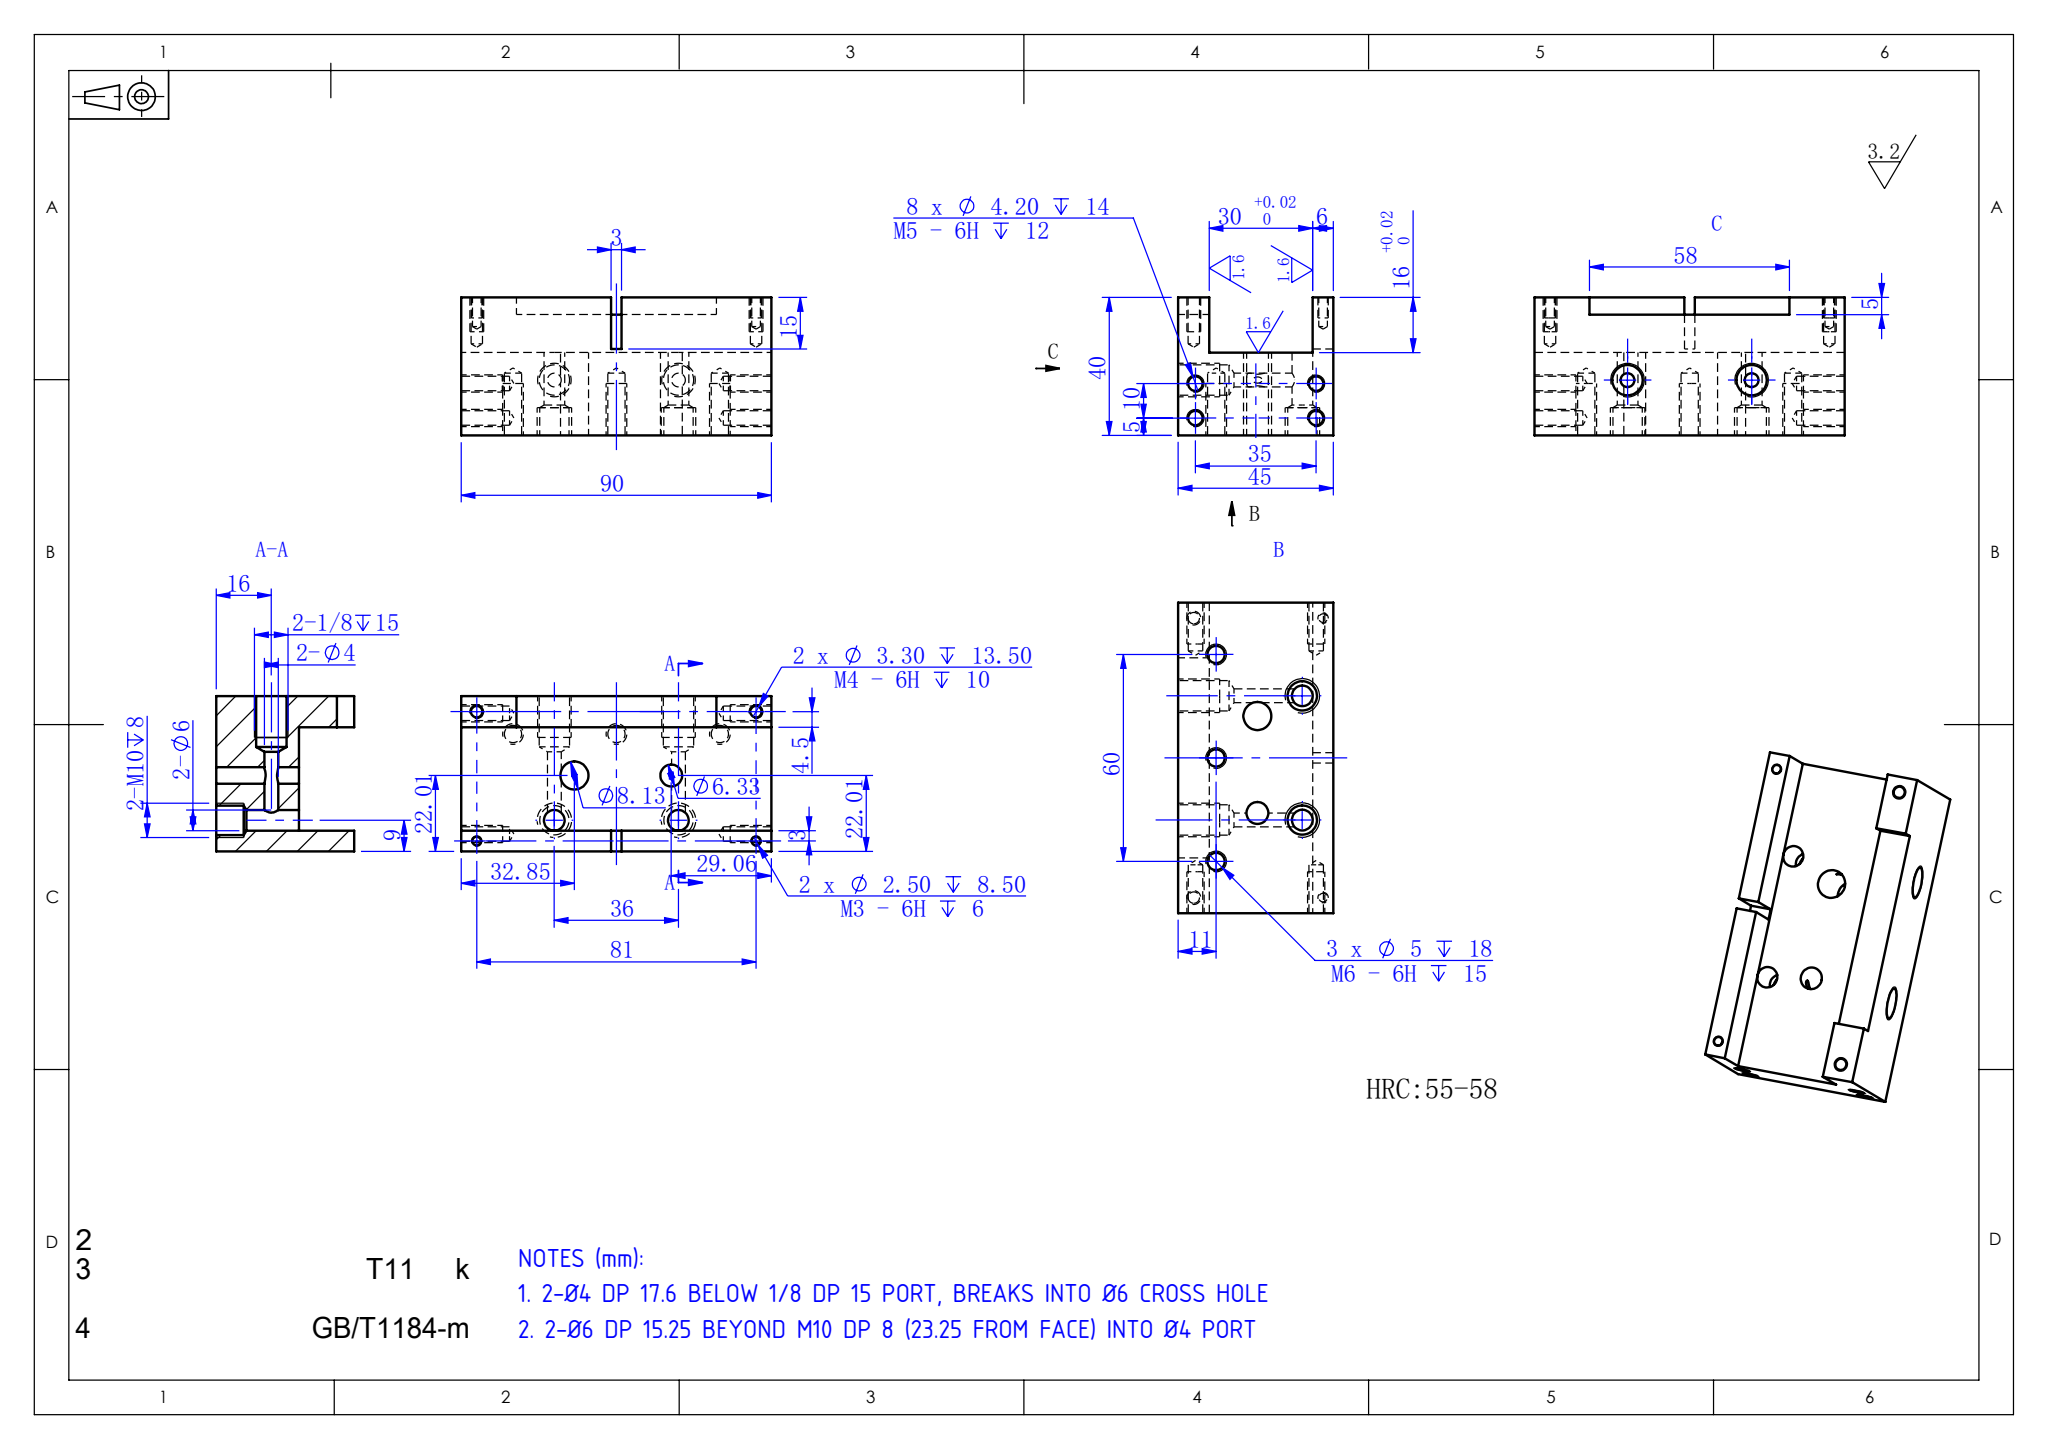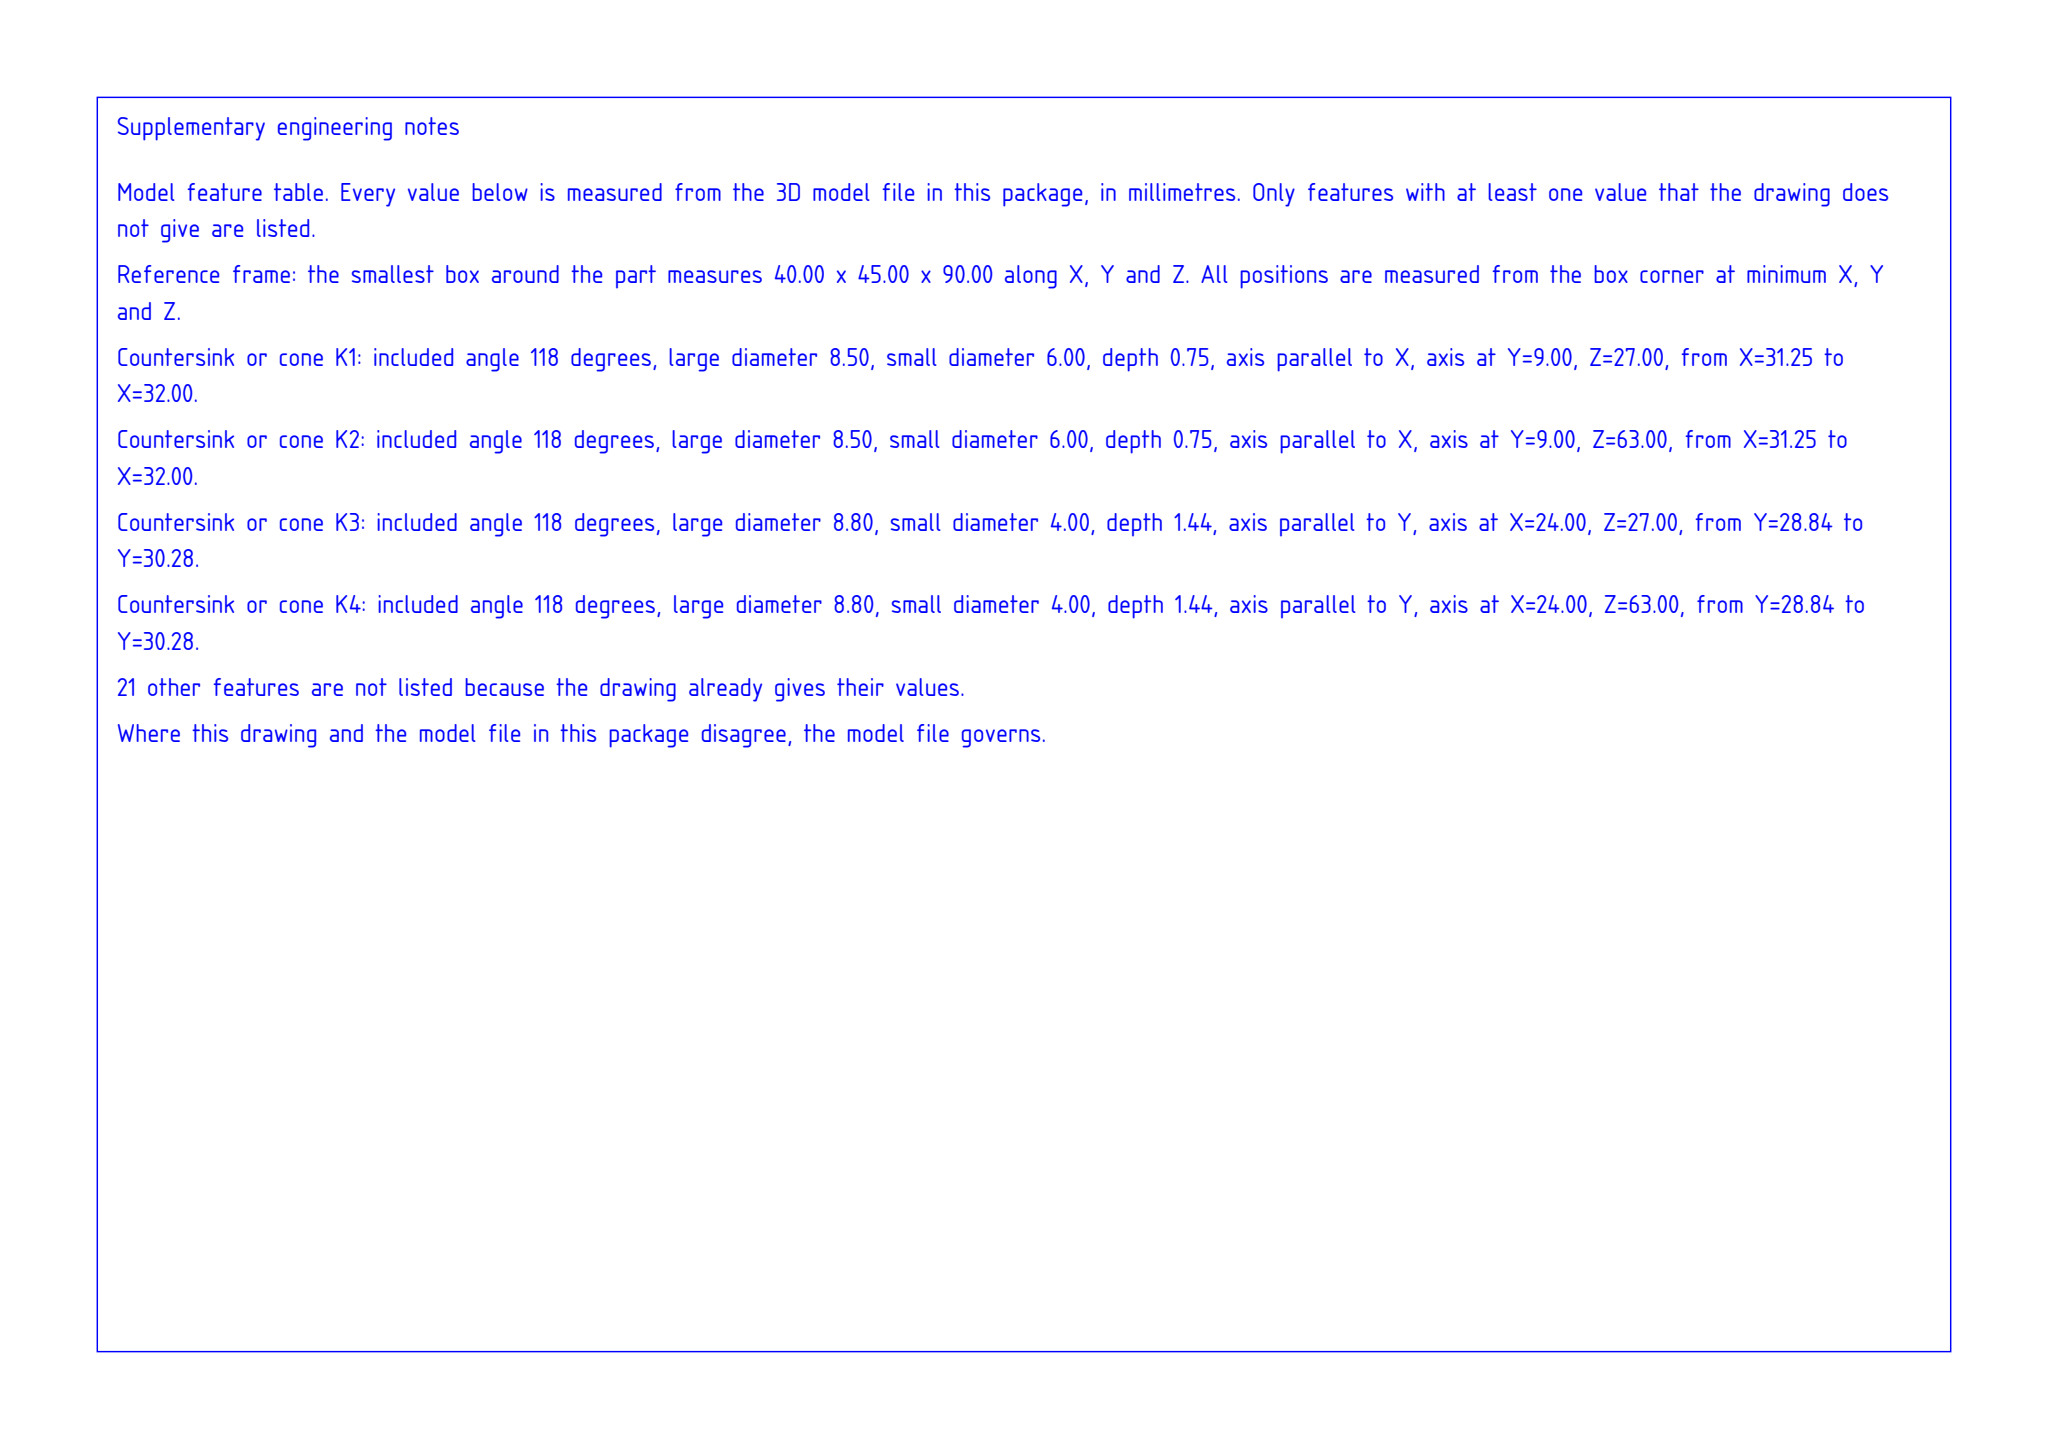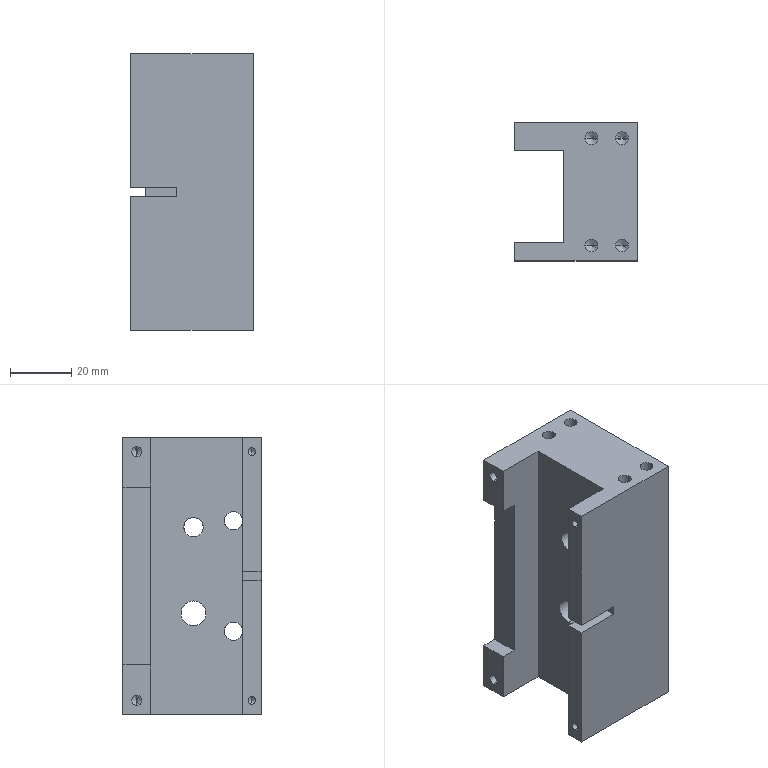Part | SolidWorks | mm | 1 solid | 106 faces | box 40 x 45 x 90 mm | volume 106811 mm3 | cylinder 50 | cone 38 | plane 18 | commonest cylinder face diameters 4.2 x16 5 x6 2.5 x4 3.3 x4 8.8 x4 4 x4 8.5 x4 6 x4
Drawing notes:
2-Ø4 DP 17.6 BELOW 1/8 DP 15 PORT, BREAKS INTO Ø6 CROSS HOLE | from the solid: cyl dia 4.0 axis y at x=24, z=27 & 63, length 17.6, below dia 8.8 y-hole (len 14.72) for 1/8 tap
2-Ø6 DP 15.25 BEYOND M10 DP 8 (23.25 FROM FACE) INTO Ø4 PORT | from the solid: cyl dia 6.0 axis x at y=9, z=27 & 63, length 15.25, following dia 8.5 x-hole length 8.0 from x=0 face; meets Ø4 at x=24
build123d program:
from build123d import *

# Parameters (mm, degrees)
SKETCH1_W                  = 40
SKETCH1_H                  = 45
BOSS_EXTRUDE1_DEPTH        = 90
SKETCH2_W                  = 16
SKETCH2_H                  = 30
CUT_EXTRUDE1_DEPTH         = 161.715
SKETCH3_W                  = 15
SKETCH3_H                  = 3
CUT_EXTRUDE2_DEPTH         = 6
SKETCH4_W                  = 58
SKETCH4_H                  = 9
CUT_EXTRUDE3_DEPTH         = 5
SKETCH5_R                  = 3
CUT_EXTRUDE4_DEPTH         = 107.791
M5_TAPPED_HOLE1_AT_2_COUNT = 2
M5_TAPPED_HOLE1_AT_2_PITCH = 35
M5_TAPPED_HOLE1_AT_3_COUNT = 2
M5_TAPPED_HOLE1_AT_3_PITCH = 36.401
M5_TAPPED_HOLE1_AT_4_COUNT = 2
M5_TAPPED_HOLE1_AT_4_PITCH = 10
M10_TAPPED_HOLE1_D         = 8.5
M10_TAPPED_HOLE1_DEPTH     = 8
M10_TAPPED_HOLE1_TIP       = 2.554
CUT_EXTRUDE6_REACH         = 160.512
SKETCH12_R                 = 2
G1_8_TAPPED_HOLE1_D        = 8.8
G1_8_TAPPED_HOLE1_DEPTH    = 14.72
G1_8_TAPPED_HOLE1_TIP      = 2.644
M4_TAPPED_HOLE1_D          = 3.3
M4_TAPPED_HOLE1_DEPTH      = 13.5
M4_TAPPED_HOLE1_TIP        = 0.9914
M3_TAPPED_HOLE1_D          = 2.5
M3_TAPPED_HOLE1_DEPTH      = 8.5
M3_TAPPED_HOLE1_TIP        = 0.7511
M6_TAPPED_HOLE1_D          = 5
M6_TAPPED_HOLE1_DEPTH      = 18
M6_TAPPED_HOLE1_TIP        = 1.502
SKETCH21_R                 = 3.165
SKETCH21_R_2               = 4.065
CUT_EXTRUDE7_DEPTH         = 62


with BuildPart() as part:
    # Sketch1 → Boss-Extrude1 (new body)
    with BuildSketch(Plane.XY):
        with Locations((-102.479, 29.734)):
            Rectangle(SKETCH1_W, SKETCH1_H)
    extrude(amount=BOSS_EXTRUDE1_DEPTH)

    # Sketch2 → Cut-Extrude1 (cut, through all)
    with BuildSketch(Plane.XY.offset(90)):
        with Locations((-114.479, 28.234)):
            Rectangle(SKETCH2_W, SKETCH2_H)
    extrude(amount=-CUT_EXTRUDE1_DEPTH, mode=Mode.SUBTRACT)

    # Sketch3 → Cut-Extrude2 (cut)
    with BuildSketch(Plane(origin=(0, 7.234, 0), x_dir=(-1, 0, 0), z_dir=(0, -1, 0))):
        with Locations((114.979, -45)):
            Rectangle(SKETCH3_W, SKETCH3_H)
    extrude(amount=-CUT_EXTRUDE2_DEPTH, mode=Mode.SUBTRACT)

    # Sketch4 → Cut-Extrude3 (cut)
    with BuildSketch(Plane.ZY.offset(122.479)):
        with Locations((45, 47.734)):
            Rectangle(SKETCH4_W, SKETCH4_H)
    extrude(amount=-CUT_EXTRUDE3_DEPTH, mode=Mode.SUBTRACT)

    # Sketch5 → Cut-Extrude4 (cut, through all)
    with BuildSketch(Plane.ZY.offset(106.479)):
        with Locations(Location((63, 16.234, 0), (0, 0, 270))):
            Circle(SKETCH5_R)
        with Locations(Location((27, 16.234, 0), (0, 0, 270))):
            Circle(SKETCH5_R)
    extrude(amount=-CUT_EXTRUDE4_DEPTH, mode=Mode.SUBTRACT)

    # Sketch6 → M5 Tapped Hole1 (revolve, cut)
    with BuildSketch(Plane(origin=(-97.479, 12.234, 90), x_dir=(0, -1, 0), z_dir=(1, 0, 0))):
        Polygon((0, 0), (0, 15.262), (2.1, 14), (2.1, 0), align=None)
    m5_tapped_hole1 = revolve(axis=Axis((-97.479, 12.234, 96.35), (0, 0, -1)), mode=Mode.SUBTRACT)

    # M5 Tapped Hole1 at 2: M5 Tapped Hole1 ×2
    with Locations(*[(0, i * M5_TAPPED_HOLE1_AT_2_PITCH, 0) for i in range(1, M5_TAPPED_HOLE1_AT_2_COUNT)]):
        add(m5_tapped_hole1, mode=Mode.SUBTRACT)

    # M5 Tapped Hole1 at 3: M5 Tapped Hole1 ×2
    with Locations(*[Vector(0.2747, 0.9615, 0) * (i * M5_TAPPED_HOLE1_AT_3_PITCH) for i in range(1, M5_TAPPED_HOLE1_AT_3_COUNT)]):
        add(m5_tapped_hole1, mode=Mode.SUBTRACT)

    # M5 Tapped Hole1 at 4: M5 Tapped Hole1 ×2
    with Locations(*[(i * M5_TAPPED_HOLE1_AT_4_PITCH, 0, 0) for i in range(1, M5_TAPPED_HOLE1_AT_4_COUNT)]):
        add(m5_tapped_hole1, mode=Mode.SUBTRACT)

    # Mirror1: M5 Tapped Hole1 across plane
    add(m5_tapped_hole1.mirror(Plane.XY.offset(45)), mode=Mode.SUBTRACT)

    # Mirror1 copy 1 sketch → Mirror1 copy 1 (revolve, cut)
    with BuildSketch(Plane(origin=(-97.479, 47.234, 0), x_dir=(0, -1, 0), z_dir=(1, 0, 0))):
        Polygon((0, 0), (0, -15.262), (2.1, -14), (2.1, 0), align=None)
    revolve(axis=Axis((-97.479, 47.234, -6.35), (0, 0, -1)), mode=Mode.SUBTRACT)

    # Mirror1 copy 2 sketch → Mirror1 copy 2 (revolve, cut)
    with BuildSketch(Plane(origin=(-87.479, 47.234, 0), x_dir=(0, -1, 0), z_dir=(1, 0, 0))):
        Polygon((0, 0), (0, -15.262), (2.1, -14), (2.1, 0), align=None)
    revolve(axis=Axis((-87.479, 47.234, -6.35), (0, 0, -1)), mode=Mode.SUBTRACT)

    # Mirror1 copy 3 sketch → Mirror1 copy 3 (revolve, cut)
    with BuildSketch(Plane(origin=(-87.479, 12.234, 0), x_dir=(0, -1, 0), z_dir=(1, 0, 0))):
        Polygon((0, 0), (0, -15.262), (2.1, -14), (2.1, 0), align=None)
    revolve(axis=Axis((-87.479, 12.234, -6.35), (0, 0, -1)), mode=Mode.SUBTRACT)

    # M10 Tapped Hole1
    with Locations(Plane(origin=(-82.479, 0, 0), x_dir=(0, 0, -1), z_dir=(1, 0, 0))):
        with Locations((-63, 16.234), (-27, 16.234)):
            Hole(M10_TAPPED_HOLE1_D / 2, depth=M10_TAPPED_HOLE1_DEPTH)
            with Locations((0, 0, -(M10_TAPPED_HOLE1_DEPTH + M10_TAPPED_HOLE1_TIP / 2))):  # 118° drill point
                Cone(0, M10_TAPPED_HOLE1_D / 2, M10_TAPPED_HOLE1_TIP, mode=Mode.SUBTRACT)

    # Sketch12 → Cut-Extrude6 (cut, up to next)
    with BuildSketch(Plane(origin=(0, 52.234, 0), x_dir=(1, 0, 0), z_dir=(0, 1, 0)), mode=Mode.PRIVATE) as cut_extrude6_sk1:
        with Locations(Location((-98.479, -63, 0), (0, 0, 270))):
            Circle(SKETCH12_R)
    cut_extrude6_tool1 = extrude(cut_extrude6_sk1.sketch, amount=-CUT_EXTRUDE6_REACH, mode=Mode.PRIVATE) & part.part
    # Sketch12 → Cut-Extrude6 (cut, up to next)
    with BuildSketch(Plane(origin=(0, 52.234, 0), x_dir=(1, 0, 0), z_dir=(0, 1, 0)), mode=Mode.PRIVATE) as cut_extrude6_sk2:
        with Locations(Location((-98.479, -27, 0), (0, 0, 270))):
            Circle(SKETCH12_R)
    cut_extrude6_tool2 = extrude(cut_extrude6_sk2.sketch, amount=-CUT_EXTRUDE6_REACH, mode=Mode.PRIVATE) & part.part
    add(cut_extrude6_tool1.solids().sort_by_distance((-98.479, 52.234, 63))[0], mode=Mode.SUBTRACT)
    add(cut_extrude6_tool2.solids().sort_by_distance((-98.479, 52.234, 27))[0], mode=Mode.SUBTRACT)

    # G1_8 Tapped Hole1
    with Locations(Plane(origin=(0, 52.234, 0), x_dir=(1, 0, 0), z_dir=(0, 1, 0))):
        with Locations((-98.479, -27), (-98.479, -63)):
            Hole(G1_8_TAPPED_HOLE1_D / 2, depth=G1_8_TAPPED_HOLE1_DEPTH)
            with Locations((0, 0, -(G1_8_TAPPED_HOLE1_DEPTH + G1_8_TAPPED_HOLE1_TIP / 2))):  # 118° drill point
                Cone(0, G1_8_TAPPED_HOLE1_D / 2, G1_8_TAPPED_HOLE1_TIP, mode=Mode.SUBTRACT)

    # M4 Tapped Hole1
    with Locations(Plane.ZY.offset(122.479)):
        with Locations((4.5, 47.734), (85.5, 47.734)):
            Hole(M4_TAPPED_HOLE1_D / 2, depth=M4_TAPPED_HOLE1_DEPTH)
            with Locations((0, 0, -(M4_TAPPED_HOLE1_DEPTH + M4_TAPPED_HOLE1_TIP / 2))):  # 118° drill point
                Cone(0, M4_TAPPED_HOLE1_D / 2, M4_TAPPED_HOLE1_TIP, mode=Mode.SUBTRACT)

    # M3 Tapped Hole1
    with Locations(Plane.ZY.offset(122.479)):
        with Locations((4.5, 10.234), (85.5, 10.234)):
            Hole(M3_TAPPED_HOLE1_D / 2, depth=M3_TAPPED_HOLE1_DEPTH)
            with Locations((0, 0, -(M3_TAPPED_HOLE1_DEPTH + M3_TAPPED_HOLE1_TIP / 2))):  # 118° drill point
                Cone(0, M3_TAPPED_HOLE1_D / 2, M3_TAPPED_HOLE1_TIP, mode=Mode.SUBTRACT)

    # M6 Tapped Hole1
    with Locations(Plane(origin=(-82.479, 0, 0), x_dir=(0, 0, -1), z_dir=(1, 0, 0))):
        with Locations((-75, 41.234), (-45, 41.234), (-15, 41.234)):
            Hole(M6_TAPPED_HOLE1_D / 2, depth=M6_TAPPED_HOLE1_DEPTH)
            with Locations((0, 0, -(M6_TAPPED_HOLE1_DEPTH + M6_TAPPED_HOLE1_TIP / 2))):  # 118° drill point
                Cone(0, M6_TAPPED_HOLE1_D / 2, M6_TAPPED_HOLE1_TIP, mode=Mode.SUBTRACT)

    # Sketch21 → Cut-Extrude7 (cut)
    with BuildSketch(Plane(origin=(-82.479, 0, 0), x_dir=(0, 0, -1), z_dir=(1, 0, 0))):
        with Locations((-60.935, 29.244)):
            Circle(SKETCH21_R)
        with Locations((-32.846, 29.244)):
            Circle(SKETCH21_R_2)
    extrude(amount=-CUT_EXTRUDE7_DEPTH, mode=Mode.SUBTRACT)


solid = part.part